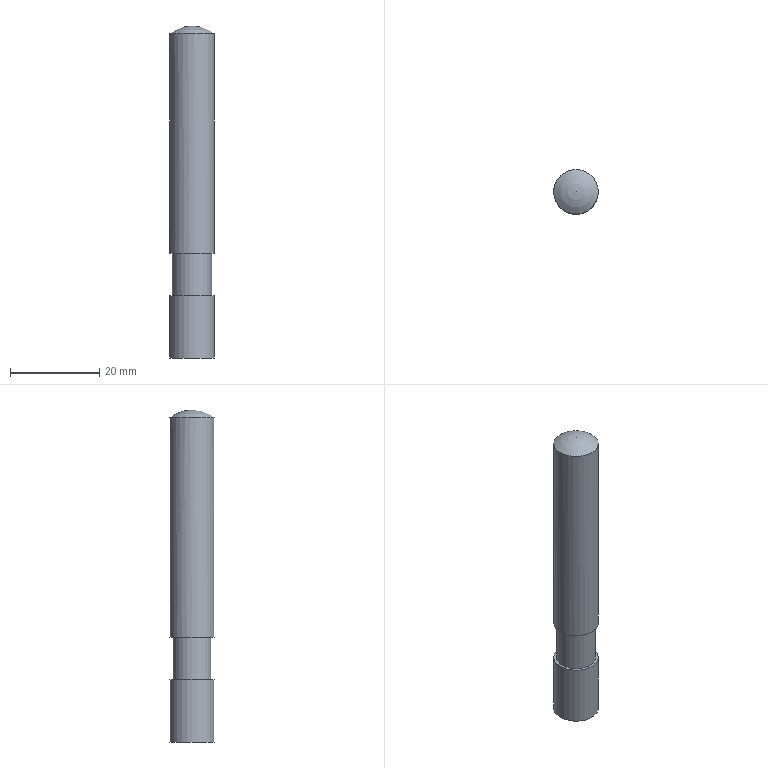Component | NX | SUPPORT_SCREW | 1 solid | 7 faces | box 10 x 10 x 74.5 mm | volume 5614 mm3 | cylinder 3 | plane 3 | sphere 1 | commonest cylinder face diameters 10 x2 8.782 x1
STEP:
#1=CARTESIAN_POINT('',(0.,0.,0.));
#2=DIRECTION('',(0.,0.,1.));
#3=DIRECTION('',(1.,0.,0.));
#4=AXIS2_PLACEMENT_3D('',#1,#2,#3);
#5=CARTESIAN_POINT('',(12.5,94.,21.5));
#6=VERTEX_POINT('',#5);
#7=CARTESIAN_POINT('',(7.5,94.,21.5));
#8=DIRECTION('',(0.,0.,-1.));
#9=DIRECTION('',(1.,0.,0.));
#10=AXIS2_PLACEMENT_3D('',#7,#8,#9);
#11=CIRCLE('',#10,5.);
#12=CARTESIAN_POINT('',(7.5,94.,72.5));
#13=DIRECTION('',(0.,0.,1.));
#14=DIRECTION('',(1.,0.,0.));
#15=AXIS2_PLACEMENT_3D('',#12,#13,#14);
#16=CYLINDRICAL_SURFACE('',#15,5.);
#17=CARTESIAN_POINT('',(6.283,-51.));
#18=DIRECTION('',(-1.,0.));
#19=VECTOR('',#18,1.);
#20=LINE('',#17,#19);
#21=(GEOMETRIC_REPRESENTATION_CONTEXT(2)PARAMETRIC_REPRESENTATION_CONTEXT()REPRESENTATION_CONTEXT('',''));
#22=DEFINITIONAL_REPRESENTATION('',(#20),#21);
#23=PCURVE('',#16,#22);
#24=CARTESIAN_POINT('',(7.5,94.,21.5));
#25=DIRECTION('',(0.,0.,1.));
#26=DIRECTION('',(1.,0.,0.));
#27=AXIS2_PLACEMENT_3D('',#24,#25,#26);
#28=PLANE('',#27);
#29=CARTESIAN_POINT('',(5.,0.));
#30=CARTESIAN_POINT('',(5.,-8.66));
#31=CARTESIAN_POINT('',(-2.5,-4.33));
#32=CARTESIAN_POINT('',(-10.,-0.));
#33=CARTESIAN_POINT('',(-2.5,4.33));
#34=CARTESIAN_POINT('',(5.,8.66));
#35=CARTESIAN_POINT('',(5.,0.));
#36=(BOUNDED_CURVE()B_SPLINE_CURVE(2,(#29,#30,#31,#32,#33,#34,#35),.UNSPECIFIED.,.T.,.F.)B_SPLINE_CURVE_WITH_KNOTS((1,2,2,2,2,1),(-2.094,0.,2.094,4.189,6.283,8.378),.UNSPECIFIED.)CURVE()GEOMETRIC_REPRESENTATION_ITEM()RATIONAL_B_SPLINE_CURVE((1.,0.5,1.,0.5,1.,0.5,1.))REPRESENTATION_ITEM(''));
#37=(GEOMETRIC_REPRESENTATION_CONTEXT(2)PARAMETRIC_REPRESENTATION_CONTEXT()REPRESENTATION_CONTEXT('',''));
#38=DEFINITIONAL_REPRESENTATION('',(#36),#37);
#39=PCURVE('',#28,#38);
#40=SURFACE_CURVE('',#11,(#23,#39),.PCURVE_S1.);
#41=EDGE_CURVE('',#6,#6,#40,.T.);
#42=ORIENTED_EDGE('',*,*,#41,.F.);
#43=CARTESIAN_POINT('',(12.5,94.,70.745));
#44=VERTEX_POINT('',#43);
#45=CARTESIAN_POINT('',(12.5,94.,21.5));
#46=CARTESIAN_POINT('',(12.5,94.,70.745));
#47=B_SPLINE_CURVE_WITH_KNOTS('',1,(#45,#46),.UNSPECIFIED.,.F.,.F.,(2,2),(-51.,-1.755),.PIECEWISE_BEZIER_KNOTS.);
#48=CARTESIAN_POINT('',(6.283,0.));
#49=DIRECTION('',(0.,1.));
#50=VECTOR('',#49,1.);
#51=LINE('',#48,#50);
#52=(GEOMETRIC_REPRESENTATION_CONTEXT(2)PARAMETRIC_REPRESENTATION_CONTEXT()REPRESENTATION_CONTEXT('',''));
#53=DEFINITIONAL_REPRESENTATION('',(#51),#52);
#54=PCURVE('',#16,#53);
#55=CARTESIAN_POINT('',(0.,0.));
#56=DIRECTION('',(0.,1.));
#57=VECTOR('',#56,1.);
#58=LINE('',#55,#57);
#59=(GEOMETRIC_REPRESENTATION_CONTEXT(2)PARAMETRIC_REPRESENTATION_CONTEXT()REPRESENTATION_CONTEXT('',''));
#60=DEFINITIONAL_REPRESENTATION('',(#58),#59);
#61=PCURVE('',#16,#60);
#62=SEAM_CURVE('',#47,(#54,#61),.PCURVE_S1.);
#63=EDGE_CURVE('',#6,#44,#62,.T.);
#64=ORIENTED_EDGE('',*,*,#63,.T.);
#65=CARTESIAN_POINT('',(7.5,99.,70.745));
#66=VERTEX_POINT('',#65);
#67=CARTESIAN_POINT('',(7.5,94.,70.745));
#68=DIRECTION('',(0.,0.,1.));
#69=DIRECTION('',(1.,0.,0.));
#70=AXIS2_PLACEMENT_3D('',#67,#68,#69);
#71=CIRCLE('',#70,5.);
#72=CARTESIAN_POINT('',(0.,-1.755));
#73=DIRECTION('',(1.,0.));
#74=VECTOR('',#73,1.);
#75=LINE('',#72,#74);
#76=(GEOMETRIC_REPRESENTATION_CONTEXT(2)PARAMETRIC_REPRESENTATION_CONTEXT()REPRESENTATION_CONTEXT('',''));
#77=DEFINITIONAL_REPRESENTATION('',(#75),#76);
#78=PCURVE('',#16,#77);
#79=CARTESIAN_POINT('',(7.5,94.,64.5));
#80=DIRECTION('',(0.,0.,1.));
#81=DIRECTION('',(0.,1.,0.));
#82=AXIS2_PLACEMENT_3D('',#79,#80,#81);
#83=SPHERICAL_SURFACE('',#82,8.);
#84=CARTESIAN_POINT('',(-1.571,0.8957));
#85=CARTESIAN_POINT('',(-1.476,0.8957));
#86=CARTESIAN_POINT('',(-1.285,0.8957));
#87=CARTESIAN_POINT('',(-0.9996,0.8957));
#88=CARTESIAN_POINT('',(-0.714,0.8957));
#89=CARTESIAN_POINT('',(-0.4284,0.8957));
#90=CARTESIAN_POINT('',(-0.1428,0.8957));
#91=CARTESIAN_POINT('',(0.1428,0.8957));
#92=CARTESIAN_POINT('',(0.4284,0.8957));
#93=CARTESIAN_POINT('',(0.714,0.8957));
#94=CARTESIAN_POINT('',(0.9996,0.8957));
#95=CARTESIAN_POINT('',(1.285,0.8957));
#96=CARTESIAN_POINT('',(1.571,0.8957));
#97=CARTESIAN_POINT('',(1.856,0.8957));
#98=CARTESIAN_POINT('',(2.142,0.8957));
#99=CARTESIAN_POINT('',(2.428,0.8957));
#100=CARTESIAN_POINT('',(2.713,0.8957));
#101=CARTESIAN_POINT('',(2.999,0.8957));
#102=CARTESIAN_POINT('',(3.284,0.8957));
#103=CARTESIAN_POINT('',(3.57,0.8957));
#104=CARTESIAN_POINT('',(3.856,0.8957));
#105=CARTESIAN_POINT('',(4.141,0.8957));
#106=CARTESIAN_POINT('',(4.427,0.8957));
#107=CARTESIAN_POINT('',(4.617,0.8957));
#108=CARTESIAN_POINT('',(4.712,0.8957));
#109=B_SPLINE_CURVE_WITH_KNOTS('',3,(#84,#85,#86,#87,#88,#89,#90,#91,#92,#93,#94,#95,#96,#97,#98,#99,#100,#101,#102,#103,#104,#105,#106,#107,#108),.UNSPECIFIED.,.F.,.F.,(4,1,1,1,1,1,1,1,1,1,1,1,1,1,1,1,1,1,1,1,1,1,4),(0.,0.2856,0.5712,0.8568,1.142,1.428,1.714,1.999,2.285,2.57,2.856,3.142,3.427,3.713,3.998,4.284,4.57,4.855,5.141,5.426,5.712,5.998,6.283),.QUASI_UNIFORM_KNOTS.);
#110=(GEOMETRIC_REPRESENTATION_CONTEXT(2)PARAMETRIC_REPRESENTATION_CONTEXT()REPRESENTATION_CONTEXT('',''));
#111=DEFINITIONAL_REPRESENTATION('',(#109),#110);
#112=PCURVE('',#83,#111);
#113=SURFACE_CURVE('',#71,(#78,#112),.PCURVE_S1.);
#114=EDGE_CURVE('',#66,#44,#113,.T.);
#115=ORIENTED_EDGE('',*,*,#114,.F.);
#116=CARTESIAN_POINT('',(7.5,94.,70.745));
#117=DIRECTION('',(0.,0.,1.));
#118=DIRECTION('',(1.,0.,0.));
#119=AXIS2_PLACEMENT_3D('',#116,#117,#118);
#120=CIRCLE('',#119,5.);
#121=CARTESIAN_POINT('',(0.,-1.755));
#122=DIRECTION('',(1.,0.));
#123=VECTOR('',#122,1.);
#124=LINE('',#121,#123);
#125=(GEOMETRIC_REPRESENTATION_CONTEXT(2)PARAMETRIC_REPRESENTATION_CONTEXT()REPRESENTATION_CONTEXT('',''));
#126=DEFINITIONAL_REPRESENTATION('',(#124),#125);
#127=PCURVE('',#16,#126);
#128=CARTESIAN_POINT('',(4.712,0.8957));
#129=CARTESIAN_POINT('',(4.808,0.8957));
#130=CARTESIAN_POINT('',(4.998,0.8957));
#131=CARTESIAN_POINT('',(5.284,0.8957));
#132=CARTESIAN_POINT('',(5.569,0.8957));
#133=CARTESIAN_POINT('',(5.855,0.8957));
#134=CARTESIAN_POINT('',(6.14,0.8957));
#135=CARTESIAN_POINT('',(6.426,0.8957));
#136=CARTESIAN_POINT('',(6.712,0.8957));
#137=CARTESIAN_POINT('',(6.997,0.8957));
#138=CARTESIAN_POINT('',(7.283,0.8957));
#139=CARTESIAN_POINT('',(7.568,0.8957));
#140=CARTESIAN_POINT('',(7.854,0.8957));
#141=CARTESIAN_POINT('',(8.14,0.8957));
#142=CARTESIAN_POINT('',(8.425,0.8957));
#143=CARTESIAN_POINT('',(8.711,0.8957));
#144=CARTESIAN_POINT('',(8.996,0.8957));
#145=CARTESIAN_POINT('',(9.282,0.8957));
#146=CARTESIAN_POINT('',(9.568,0.8957));
#147=CARTESIAN_POINT('',(9.853,0.8957));
#148=CARTESIAN_POINT('',(10.139,0.8957));
#149=CARTESIAN_POINT('',(10.424,0.8957));
#150=CARTESIAN_POINT('',(10.71,0.8957));
#151=CARTESIAN_POINT('',(10.9,0.8957));
#152=CARTESIAN_POINT('',(10.996,0.8957));
#153=B_SPLINE_CURVE_WITH_KNOTS('',3,(#128,#129,#130,#131,#132,#133,#134,#135,#136,#137,#138,#139,#140,#141,#142,#143,#144,#145,#146,#147,#148,#149,#150,#151,#152),.UNSPECIFIED.,.F.,.F.,(4,1,1,1,1,1,1,1,1,1,1,1,1,1,1,1,1,1,1,1,1,1,4),(0.,0.2856,0.5712,0.8568,1.142,1.428,1.714,1.999,2.285,2.57,2.856,3.142,3.427,3.713,3.998,4.284,4.57,4.855,5.141,5.426,5.712,5.998,6.283),.QUASI_UNIFORM_KNOTS.);
#154=(GEOMETRIC_REPRESENTATION_CONTEXT(2)PARAMETRIC_REPRESENTATION_CONTEXT()REPRESENTATION_CONTEXT('',''));
#155=DEFINITIONAL_REPRESENTATION('',(#153),#154);
#156=PCURVE('',#83,#155);
#157=SURFACE_CURVE('',#120,(#127,#156),.PCURVE_S1.);
#158=EDGE_CURVE('',#44,#66,#157,.T.);
#159=ORIENTED_EDGE('',*,*,#158,.F.);
#160=ORIENTED_EDGE('',*,*,#63,.F.);
#161=EDGE_LOOP('',(#42,#64,#115,#159,#160));
#162=FACE_BOUND('',#161,.T.);
#163=ADVANCED_FACE('',(#162),#16,.T.);
#164=ORIENTED_EDGE('',*,*,#158,.T.);
#165=CARTESIAN_POINT('',(7.5,94.,72.5));
#166=VERTEX_POINT('',#165);
#167=CARTESIAN_POINT('',(7.5,99.,70.745));
#168=CARTESIAN_POINT('',(7.5,98.157,71.42));
#169=CARTESIAN_POINT('',(7.5,97.2,71.953));
#170=CARTESIAN_POINT('',(7.5,96.16,72.318));
#171=CARTESIAN_POINT('',(7.5,95.08,72.5));
#172=CARTESIAN_POINT('',(7.5,94.,72.5));
#173=B_SPLINE_CURVE_WITH_KNOTS('',5,(#167,#168,#169,#170,#171,#172),.UNSPECIFIED.,.F.,.F.,(6,6),(0.8957,1.571),.PIECEWISE_BEZIER_KNOTS.);
#174=CARTESIAN_POINT('',(6.283,0.));
#175=DIRECTION('',(0.,1.));
#176=VECTOR('',#175,1.);
#177=LINE('',#174,#176);
#178=(GEOMETRIC_REPRESENTATION_CONTEXT(2)PARAMETRIC_REPRESENTATION_CONTEXT()REPRESENTATION_CONTEXT('',''));
#179=DEFINITIONAL_REPRESENTATION('',(#177),#178);
#180=PCURVE('',#83,#179);
#181=CARTESIAN_POINT('',(0.,0.));
#182=DIRECTION('',(0.,1.));
#183=VECTOR('',#182,1.);
#184=LINE('',#181,#183);
#185=(GEOMETRIC_REPRESENTATION_CONTEXT(2)PARAMETRIC_REPRESENTATION_CONTEXT()REPRESENTATION_CONTEXT('',''));
#186=DEFINITIONAL_REPRESENTATION('',(#184),#185);
#187=PCURVE('',#83,#186);
#188=SEAM_CURVE('',#173,(#180,#187),.PCURVE_S1.);
#189=EDGE_CURVE('',#66,#166,#188,.T.);
#190=ORIENTED_EDGE('',*,*,#189,.T.);
#191=ORIENTED_EDGE('',*,*,#189,.F.);
#192=ORIENTED_EDGE('',*,*,#114,.T.);
#193=EDGE_LOOP('',(#164,#190,#191,#192));
#194=FACE_BOUND('',#193,.T.);
#195=ADVANCED_FACE('',(#194),#83,.T.);
#196=CARTESIAN_POINT('',(11.891,94.,21.5));
#197=VERTEX_POINT('',#196);
#198=CARTESIAN_POINT('',(7.5,94.,21.5));
#199=DIRECTION('',(0.,0.,-1.));
#200=DIRECTION('',(1.,0.,0.));
#201=AXIS2_PLACEMENT_3D('',#198,#199,#200);
#202=CIRCLE('',#201,4.391);
#203=CARTESIAN_POINT('',(7.5,94.,21.5));
#204=DIRECTION('',(0.,0.,-1.));
#205=DIRECTION('',(-1.,0.,0.));
#206=AXIS2_PLACEMENT_3D('',#203,#204,#205);
#207=CYLINDRICAL_SURFACE('',#206,4.391);
#208=CARTESIAN_POINT('',(3.142,0.));
#209=DIRECTION('',(1.,0.));
#210=VECTOR('',#209,1.);
#211=LINE('',#208,#210);
#212=(GEOMETRIC_REPRESENTATION_CONTEXT(2)PARAMETRIC_REPRESENTATION_CONTEXT()REPRESENTATION_CONTEXT('',''));
#213=DEFINITIONAL_REPRESENTATION('',(#211),#212);
#214=PCURVE('',#207,#213);
#215=CARTESIAN_POINT('',(4.391,0.));
#216=CARTESIAN_POINT('',(4.391,-7.606));
#217=CARTESIAN_POINT('',(-2.196,-3.803));
#218=CARTESIAN_POINT('',(-8.782,-0.));
#219=CARTESIAN_POINT('',(-2.196,3.803));
#220=CARTESIAN_POINT('',(4.391,7.606));
#221=CARTESIAN_POINT('',(4.391,0.));
#222=(BOUNDED_CURVE()B_SPLINE_CURVE(2,(#215,#216,#217,#218,#219,#220,#221),.UNSPECIFIED.,.T.,.F.)B_SPLINE_CURVE_WITH_KNOTS((1,2,2,2,2,1),(-2.094,0.,2.094,4.189,6.283,8.378),.UNSPECIFIED.)CURVE()GEOMETRIC_REPRESENTATION_ITEM()RATIONAL_B_SPLINE_CURVE((1.,0.5,1.,0.5,1.,0.5,1.))REPRESENTATION_ITEM(''));
#223=(GEOMETRIC_REPRESENTATION_CONTEXT(2)PARAMETRIC_REPRESENTATION_CONTEXT()REPRESENTATION_CONTEXT('',''));
#224=DEFINITIONAL_REPRESENTATION('',(#222),#223);
#225=PCURVE('',#28,#224);
#226=SURFACE_CURVE('',#202,(#214,#225),.PCURVE_S1.);
#227=EDGE_CURVE('',#197,#197,#226,.T.);
#228=ORIENTED_EDGE('',*,*,#227,.T.);
#229=CARTESIAN_POINT('',(11.891,94.,12.));
#230=VERTEX_POINT('',#229);
#231=CARTESIAN_POINT('',(11.891,94.,21.5));
#232=CARTESIAN_POINT('',(11.891,94.,12.));
#233=B_SPLINE_CURVE_WITH_KNOTS('',1,(#231,#232),.UNSPECIFIED.,.F.,.F.,(2,2),(0.,9.5),.PIECEWISE_BEZIER_KNOTS.);
#234=CARTESIAN_POINT('',(9.425,0.));
#235=DIRECTION('',(0.,1.));
#236=VECTOR('',#235,1.);
#237=LINE('',#234,#236);
#238=(GEOMETRIC_REPRESENTATION_CONTEXT(2)PARAMETRIC_REPRESENTATION_CONTEXT()REPRESENTATION_CONTEXT('',''));
#239=DEFINITIONAL_REPRESENTATION('',(#237),#238);
#240=PCURVE('',#207,#239);
#241=CARTESIAN_POINT('',(3.142,0.));
#242=DIRECTION('',(0.,1.));
#243=VECTOR('',#242,1.);
#244=LINE('',#241,#243);
#245=(GEOMETRIC_REPRESENTATION_CONTEXT(2)PARAMETRIC_REPRESENTATION_CONTEXT()REPRESENTATION_CONTEXT('',''));
#246=DEFINITIONAL_REPRESENTATION('',(#244),#245);
#247=PCURVE('',#207,#246);
#248=SEAM_CURVE('',#233,(#240,#247),.PCURVE_S1.);
#249=EDGE_CURVE('',#197,#230,#248,.T.);
#250=ORIENTED_EDGE('',*,*,#249,.T.);
#251=CARTESIAN_POINT('',(7.5,94.,12.));
#252=DIRECTION('',(0.,0.,-1.));
#253=DIRECTION('',(1.,0.,0.));
#254=AXIS2_PLACEMENT_3D('',#251,#252,#253);
#255=CIRCLE('',#254,4.391);
#256=CARTESIAN_POINT('',(3.142,9.5));
#257=DIRECTION('',(1.,0.));
#258=VECTOR('',#257,1.);
#259=LINE('',#256,#258);
#260=(GEOMETRIC_REPRESENTATION_CONTEXT(2)PARAMETRIC_REPRESENTATION_CONTEXT()REPRESENTATION_CONTEXT('',''));
#261=DEFINITIONAL_REPRESENTATION('',(#259),#260);
#262=PCURVE('',#207,#261);
#263=CARTESIAN_POINT('',(7.5,94.,12.));
#264=DIRECTION('',(0.,0.,1.));
#265=DIRECTION('',(1.,0.,0.));
#266=AXIS2_PLACEMENT_3D('',#263,#264,#265);
#267=PLANE('',#266);
#268=CARTESIAN_POINT('',(4.391,0.));
#269=CARTESIAN_POINT('',(4.391,-7.606));
#270=CARTESIAN_POINT('',(-2.196,-3.803));
#271=CARTESIAN_POINT('',(-8.782,-0.));
#272=CARTESIAN_POINT('',(-2.196,3.803));
#273=CARTESIAN_POINT('',(4.391,7.606));
#274=CARTESIAN_POINT('',(4.391,0.));
#275=(BOUNDED_CURVE()B_SPLINE_CURVE(2,(#268,#269,#270,#271,#272,#273,#274),.UNSPECIFIED.,.T.,.F.)B_SPLINE_CURVE_WITH_KNOTS((1,2,2,2,2,1),(-2.094,0.,2.094,4.189,6.283,8.378),.UNSPECIFIED.)CURVE()GEOMETRIC_REPRESENTATION_ITEM()RATIONAL_B_SPLINE_CURVE((1.,0.5,1.,0.5,1.,0.5,1.))REPRESENTATION_ITEM(''));
#276=(GEOMETRIC_REPRESENTATION_CONTEXT(2)PARAMETRIC_REPRESENTATION_CONTEXT()REPRESENTATION_CONTEXT('',''));
#277=DEFINITIONAL_REPRESENTATION('',(#275),#276);
#278=PCURVE('',#267,#277);
#279=SURFACE_CURVE('',#255,(#262,#278),.PCURVE_S1.);
#280=EDGE_CURVE('',#230,#230,#279,.T.);
#281=ORIENTED_EDGE('',*,*,#280,.F.);
#282=ORIENTED_EDGE('',*,*,#249,.F.);
#283=EDGE_LOOP('',(#228,#250,#281,#282));
#284=FACE_BOUND('',#283,.T.);
#285=ADVANCED_FACE('',(#284),#207,.T.);
#286=ORIENTED_EDGE('',*,*,#41,.T.);
#287=EDGE_LOOP('',(#286));
#288=FACE_BOUND('',#287,.T.);
#289=ORIENTED_EDGE('',*,*,#227,.F.);
#290=EDGE_LOOP('',(#289));
#291=FACE_BOUND('',#290,.T.);
#292=ADVANCED_FACE('',(#288,#291),#28,.F.);
#293=CARTESIAN_POINT('',(12.5,94.,12.));
#294=VERTEX_POINT('',#293);
#295=CARTESIAN_POINT('',(7.5,94.,12.));
#296=DIRECTION('',(0.,0.,-1.));
#297=DIRECTION('',(1.,0.,0.));
#298=AXIS2_PLACEMENT_3D('',#295,#296,#297);
#299=CIRCLE('',#298,5.);
#300=CARTESIAN_POINT('',(5.,0.));
#301=CARTESIAN_POINT('',(5.,-8.66));
#302=CARTESIAN_POINT('',(-2.5,-4.33));
#303=CARTESIAN_POINT('',(-10.,-0.));
#304=CARTESIAN_POINT('',(-2.5,4.33));
#305=CARTESIAN_POINT('',(5.,8.66));
#306=CARTESIAN_POINT('',(5.,0.));
#307=(BOUNDED_CURVE()B_SPLINE_CURVE(2,(#300,#301,#302,#303,#304,#305,#306),.UNSPECIFIED.,.T.,.F.)B_SPLINE_CURVE_WITH_KNOTS((1,2,2,2,2,1),(-2.094,0.,2.094,4.189,6.283,8.378),.UNSPECIFIED.)CURVE()GEOMETRIC_REPRESENTATION_ITEM()RATIONAL_B_SPLINE_CURVE((1.,0.5,1.,0.5,1.,0.5,1.))REPRESENTATION_ITEM(''));
#308=(GEOMETRIC_REPRESENTATION_CONTEXT(2)PARAMETRIC_REPRESENTATION_CONTEXT()REPRESENTATION_CONTEXT('',''));
#309=DEFINITIONAL_REPRESENTATION('',(#307),#308);
#310=PCURVE('',#267,#309);
#311=CARTESIAN_POINT('',(7.5,94.,72.5));
#312=DIRECTION('',(0.,0.,1.));
#313=DIRECTION('',(1.,0.,0.));
#314=AXIS2_PLACEMENT_3D('',#311,#312,#313);
#315=CYLINDRICAL_SURFACE('',#314,5.);
#316=CARTESIAN_POINT('',(6.283,-60.5));
#317=DIRECTION('',(-1.,0.));
#318=VECTOR('',#317,1.);
#319=LINE('',#316,#318);
#320=(GEOMETRIC_REPRESENTATION_CONTEXT(2)PARAMETRIC_REPRESENTATION_CONTEXT()REPRESENTATION_CONTEXT('',''));
#321=DEFINITIONAL_REPRESENTATION('',(#319),#320);
#322=PCURVE('',#315,#321);
#323=SURFACE_CURVE('',#299,(#310,#322),.PCURVE_S1.);
#324=EDGE_CURVE('',#294,#294,#323,.T.);
#325=ORIENTED_EDGE('',*,*,#324,.F.);
#326=EDGE_LOOP('',(#325));
#327=FACE_BOUND('',#326,.T.);
#328=ORIENTED_EDGE('',*,*,#280,.T.);
#329=EDGE_LOOP('',(#328));
#330=FACE_BOUND('',#329,.T.);
#331=ADVANCED_FACE('',(#327,#330),#267,.T.);
#332=CARTESIAN_POINT('',(12.5,94.,-2.));
#333=VERTEX_POINT('',#332);
#334=CARTESIAN_POINT('',(7.5,94.,-2.));
#335=DIRECTION('',(0.,0.,1.));
#336=DIRECTION('',(1.,0.,0.));
#337=AXIS2_PLACEMENT_3D('',#334,#335,#336);
#338=CIRCLE('',#337,5.);
#339=CARTESIAN_POINT('',(7.5,94.,-2.));
#340=DIRECTION('',(0.,0.,1.));
#341=DIRECTION('',(1.,0.,0.));
#342=AXIS2_PLACEMENT_3D('',#339,#340,#341);
#343=PLANE('',#342);
#344=CARTESIAN_POINT('',(0.,0.));
#345=DIRECTION('',(1.,0.));
#346=AXIS2_PLACEMENT_2D('',#344,#345);
#347=CIRCLE('',#346,5.);
#348=(GEOMETRIC_REPRESENTATION_CONTEXT(2)PARAMETRIC_REPRESENTATION_CONTEXT()REPRESENTATION_CONTEXT('',''));
#349=DEFINITIONAL_REPRESENTATION('',(#347),#348);
#350=PCURVE('',#343,#349);
#351=CARTESIAN_POINT('',(0.,-74.5));
#352=DIRECTION('',(1.,0.));
#353=VECTOR('',#352,1.);
#354=LINE('',#351,#353);
#355=(GEOMETRIC_REPRESENTATION_CONTEXT(2)PARAMETRIC_REPRESENTATION_CONTEXT()REPRESENTATION_CONTEXT('',''));
#356=DEFINITIONAL_REPRESENTATION('',(#354),#355);
#357=PCURVE('',#315,#356);
#358=SURFACE_CURVE('',#338,(#350,#357),.PCURVE_S1.);
#359=EDGE_CURVE('',#333,#333,#358,.T.);
#360=ORIENTED_EDGE('',*,*,#359,.F.);
#361=EDGE_LOOP('',(#360));
#362=FACE_BOUND('',#361,.T.);
#363=ADVANCED_FACE('',(#362),#343,.F.);
#364=ORIENTED_EDGE('',*,*,#359,.T.);
#365=CARTESIAN_POINT('',(12.5,94.,-2.));
#366=CARTESIAN_POINT('',(12.5,94.,12.));
#367=B_SPLINE_CURVE_WITH_KNOTS('',1,(#365,#366),.UNSPECIFIED.,.F.,.F.,(2,2),(-74.5,-60.5),.PIECEWISE_BEZIER_KNOTS.);
#368=CARTESIAN_POINT('',(6.283,0.));
#369=DIRECTION('',(0.,1.));
#370=VECTOR('',#369,1.);
#371=LINE('',#368,#370);
#372=(GEOMETRIC_REPRESENTATION_CONTEXT(2)PARAMETRIC_REPRESENTATION_CONTEXT()REPRESENTATION_CONTEXT('',''));
#373=DEFINITIONAL_REPRESENTATION('',(#371),#372);
#374=PCURVE('',#315,#373);
#375=CARTESIAN_POINT('',(0.,0.));
#376=DIRECTION('',(0.,1.));
#377=VECTOR('',#376,1.);
#378=LINE('',#375,#377);
#379=(GEOMETRIC_REPRESENTATION_CONTEXT(2)PARAMETRIC_REPRESENTATION_CONTEXT()REPRESENTATION_CONTEXT('',''));
#380=DEFINITIONAL_REPRESENTATION('',(#378),#379);
#381=PCURVE('',#315,#380);
#382=SEAM_CURVE('',#367,(#374,#381),.PCURVE_S1.);
#383=EDGE_CURVE('',#333,#294,#382,.T.);
#384=ORIENTED_EDGE('',*,*,#383,.T.);
#385=ORIENTED_EDGE('',*,*,#324,.T.);
#386=ORIENTED_EDGE('',*,*,#383,.F.);
#387=EDGE_LOOP('',(#364,#384,#385,#386));
#388=FACE_BOUND('',#387,.T.);
#389=ADVANCED_FACE('',(#388),#315,.T.);
#390=CLOSED_SHELL('',(#163,#195,#285,#292,#331,#363,#389));
#391=MANIFOLD_SOLID_BREP('',#390);
#392=(LENGTH_UNIT()NAMED_UNIT(*)SI_UNIT(.MILLI.,.METRE.));
#393=UNCERTAINTY_MEASURE_WITH_UNIT(LENGTH_MEASURE(0.00001),#392,'','');
#394=(NAMED_UNIT(*)PLANE_ANGLE_UNIT()SI_UNIT($,.RADIAN.));
#395=(NAMED_UNIT(*)SI_UNIT($,.STERADIAN.)SOLID_ANGLE_UNIT());
#396=(GEOMETRIC_REPRESENTATION_CONTEXT(3)GLOBAL_UNCERTAINTY_ASSIGNED_CONTEXT((#393))GLOBAL_UNIT_ASSIGNED_CONTEXT((#392,#394,#395))REPRESENTATION_CONTEXT('',''));
#397=ADVANCED_BREP_SHAPE_REPRESENTATION('',(#4,#391),#396);